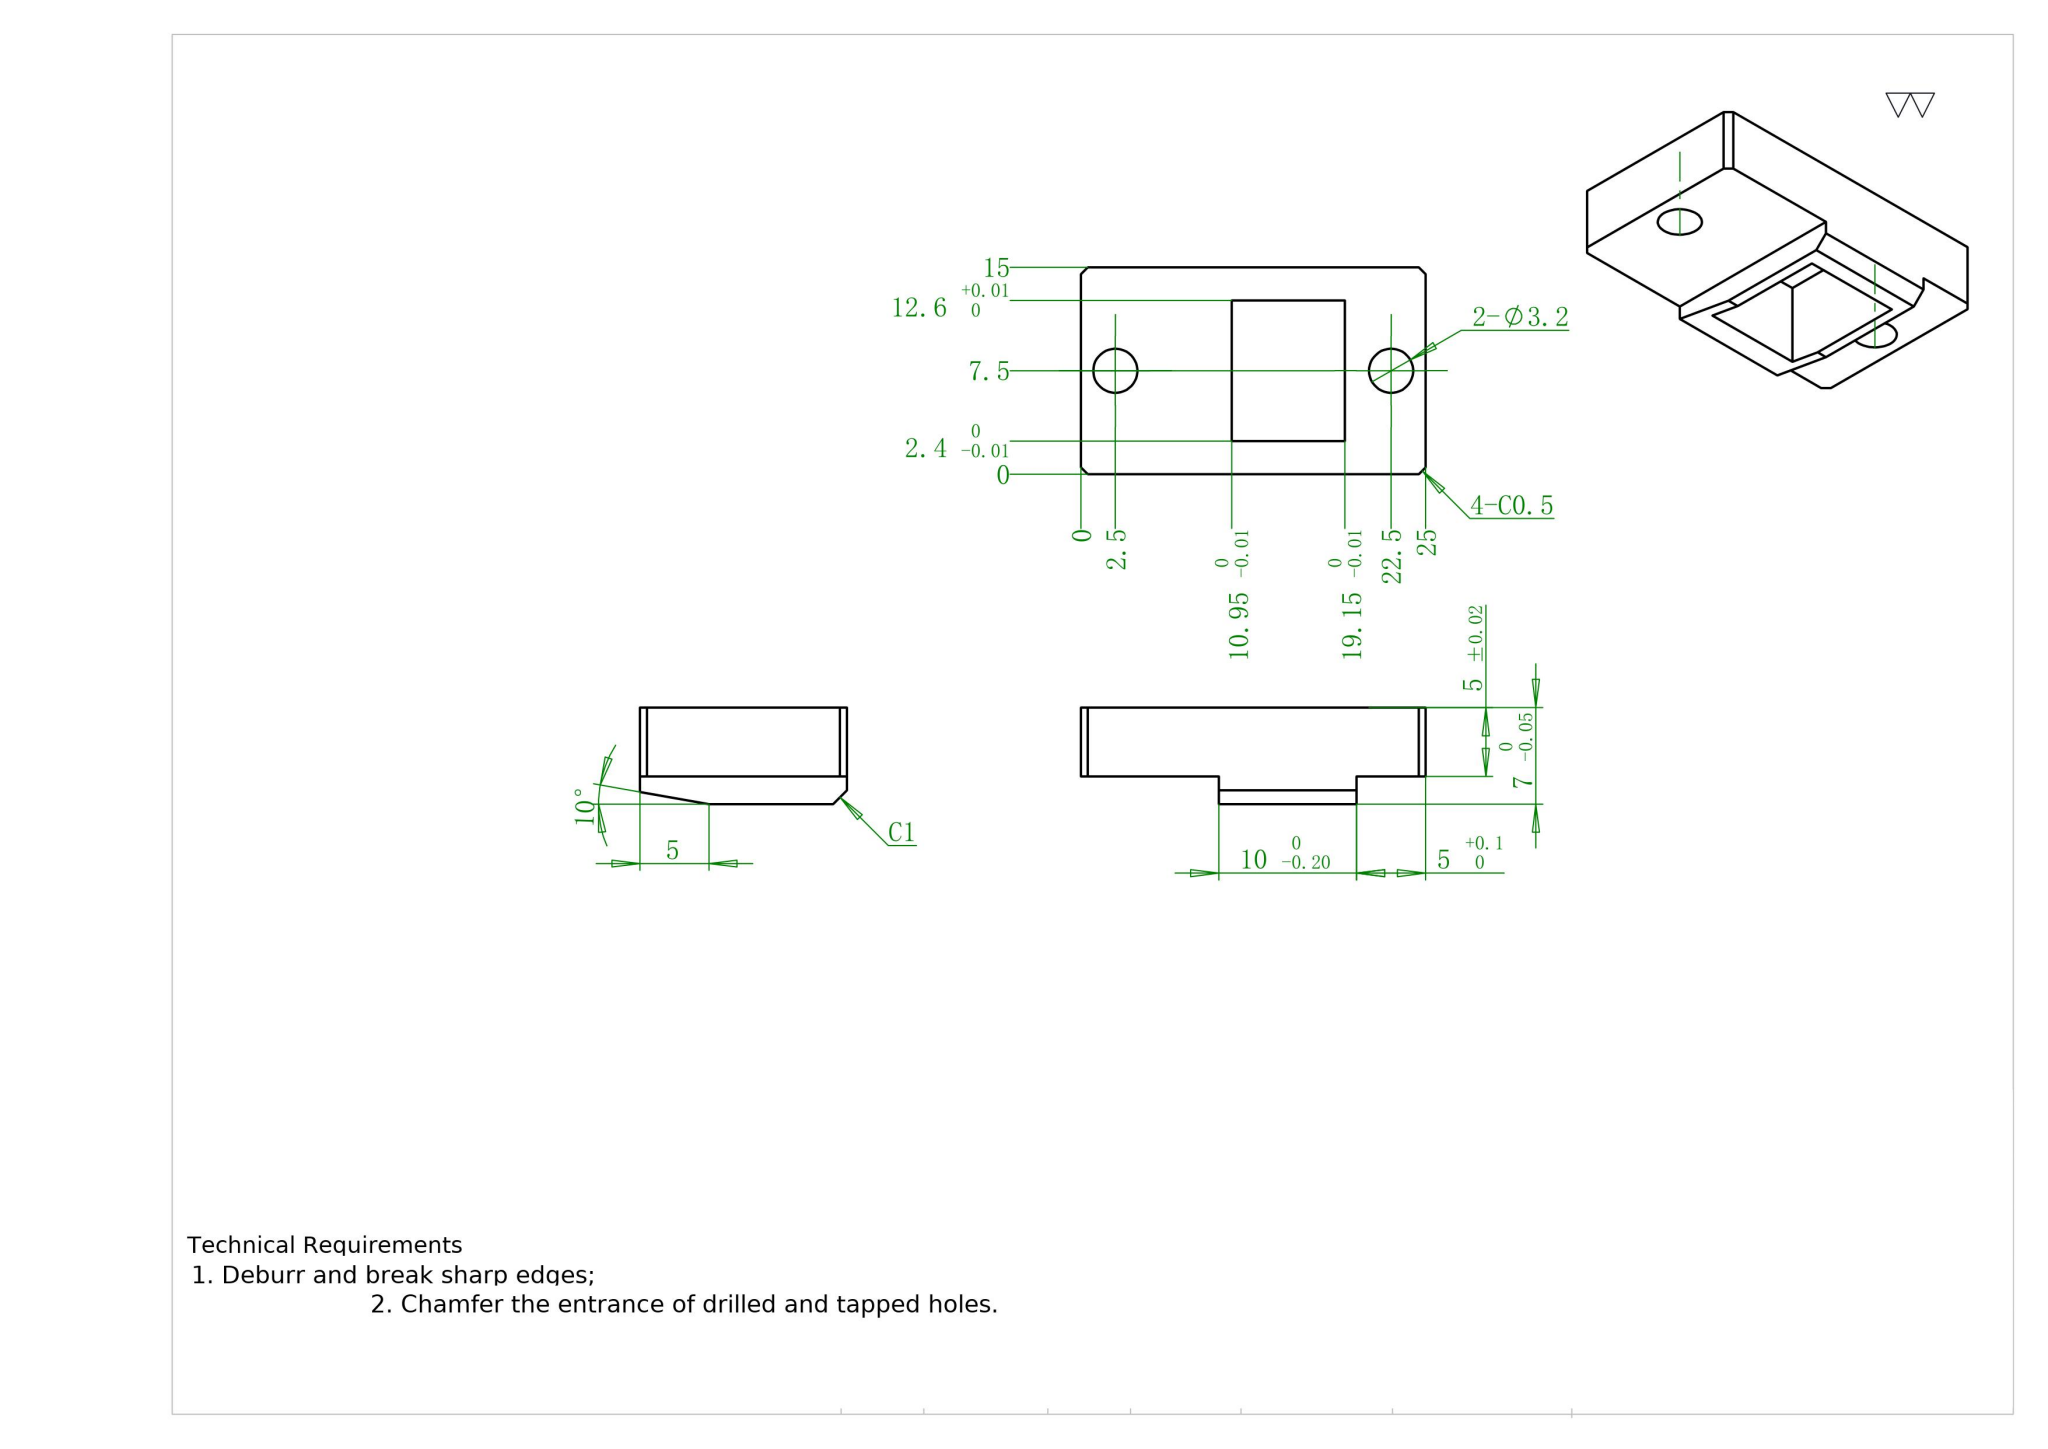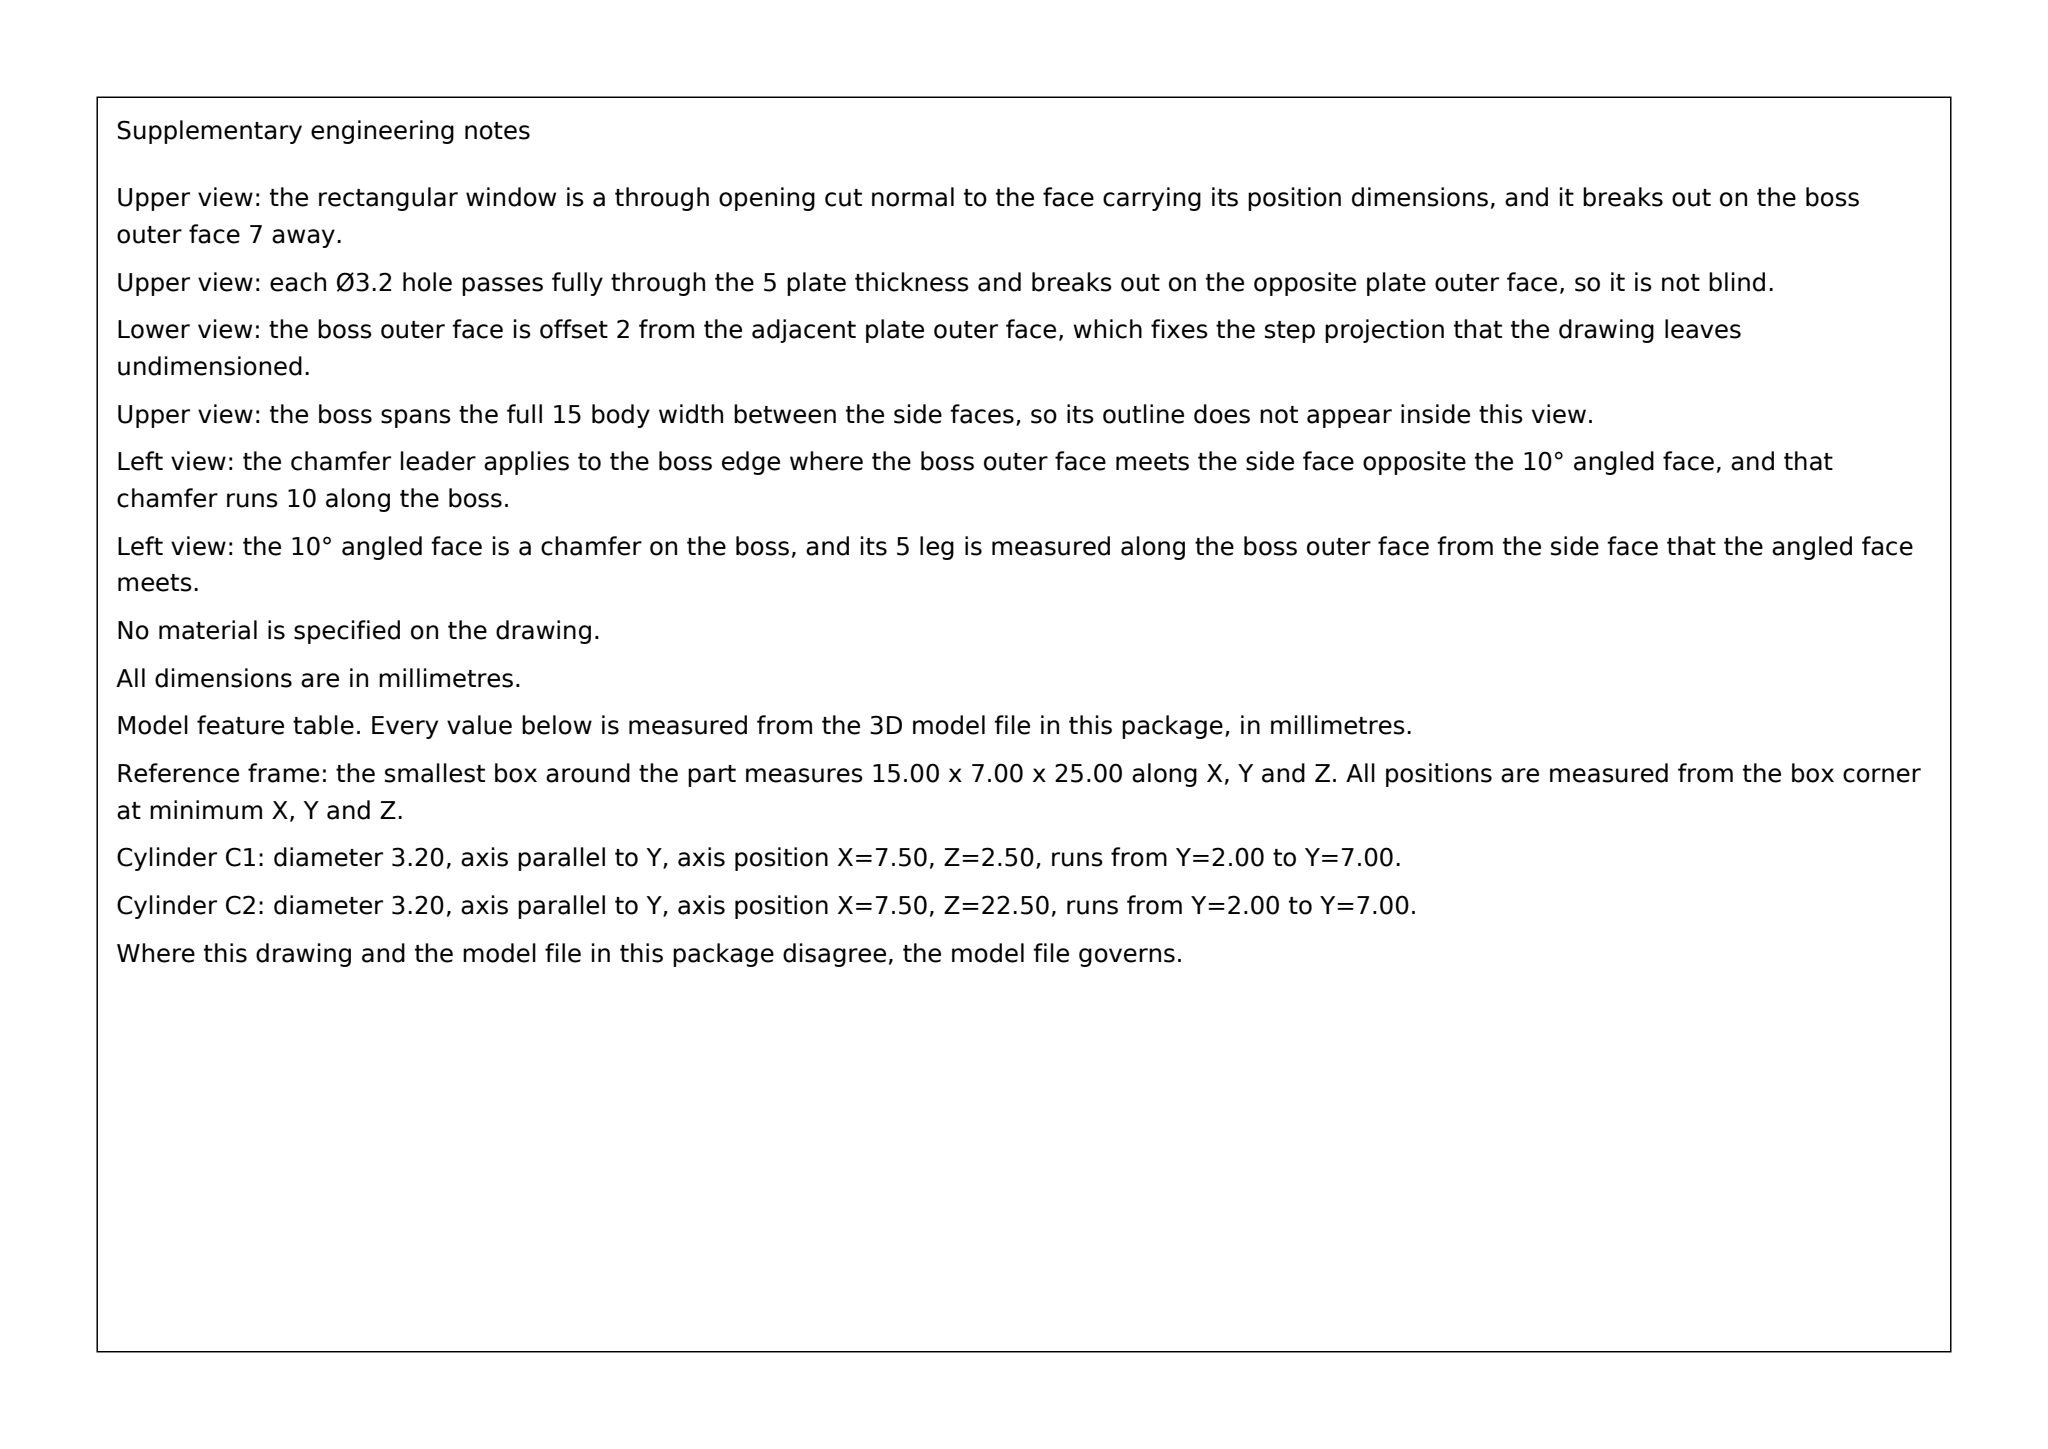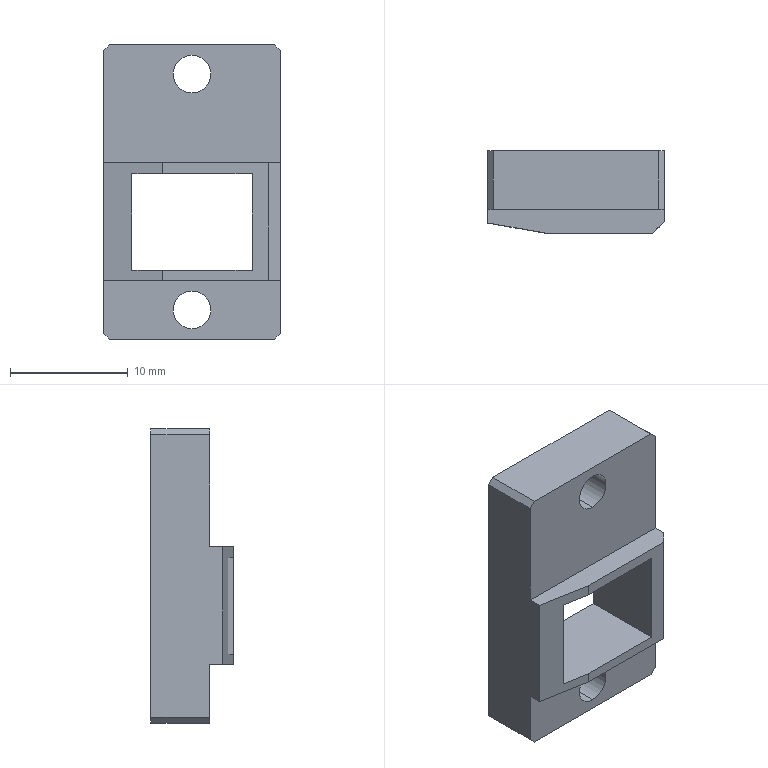Part | SolidWorks | mm | 1 solid | 24 faces | box 15 x 7 x 25 mm | volume 1484 mm3 | plane 20 | cylinder 4 | commonest cylinder face diameters 3.2 x4
Drawing notes:
2-Ø3.2 DP 5 (BLIND, FROM TOP FACE) | from the solid: cylinders dia 3.2, axis y, length 5.0 at z=2.5 and z=22.5, bbox y=7.0 so holes start at top face y=7 and end at y=2.0 (y-plane 2.0 count 2)
STEP:
#1=CARTESIAN_POINT('',(0.,-2.5,0.9));
#2=VERTEX_POINT('',#1);
#3=CARTESIAN_POINT('',(0.,-2.5,4.1));
#4=VERTEX_POINT('',#3);
#5=CARTESIAN_POINT('',(0.,-2.5,2.5));
#6=DIRECTION('',(0.,1.,0.));
#7=DIRECTION('',(0.,0.,1.));
#8=AXIS2_PLACEMENT_3D('',#5,#6,#7);
#9=CIRCLE('',#8,1.6);
#10=EDGE_CURVE('',#2,#4,#9,.T.);
#11=ORIENTED_EDGE('',*,*,#10,.F.);
#12=CARTESIAN_POINT('',(0.,2.5,0.9));
#13=VERTEX_POINT('',#12);
#14=CARTESIAN_POINT('',(0.,2.5,0.9));
#15=DIRECTION('',(0.,1.,0.));
#16=VECTOR('',#15,1000.);
#17=LINE('',#14,#16);
#18=EDGE_CURVE('',#2,#13,#17,.T.);
#19=ORIENTED_EDGE('',*,*,#18,.T.);
#20=CARTESIAN_POINT('',(0.,2.5,4.1));
#21=VERTEX_POINT('',#20);
#22=CARTESIAN_POINT('',(0.,2.5,2.5));
#23=DIRECTION('',(0.,1.,0.));
#24=DIRECTION('',(0.,0.,1.));
#25=AXIS2_PLACEMENT_3D('',#22,#23,#24);
#26=CIRCLE('',#25,1.6);
#27=EDGE_CURVE('',#13,#21,#26,.T.);
#28=ORIENTED_EDGE('',*,*,#27,.T.);
#29=CARTESIAN_POINT('',(0.,2.5,4.1));
#30=DIRECTION('',(0.,1.,0.));
#31=VECTOR('',#30,1000.);
#32=LINE('',#29,#31);
#33=EDGE_CURVE('',#4,#21,#32,.T.);
#34=ORIENTED_EDGE('',*,*,#33,.F.);
#35=EDGE_LOOP('',(#11,#19,#28,#34));
#36=FACE_OUTER_BOUND('',#35,.T.);
#37=CARTESIAN_POINT('',(0.,2.5,2.5));
#38=DIRECTION('',(0.,1.,0.));
#39=DIRECTION('',(0.,0.,1.));
#40=AXIS2_PLACEMENT_3D('',#37,#38,#39);
#41=CYLINDRICAL_SURFACE('',#40,1.6);
#42=ADVANCED_FACE('',(#36),#41,.F.);
#43=CARTESIAN_POINT('',(0.,-2.5,20.9));
#44=VERTEX_POINT('',#43);
#45=CARTESIAN_POINT('',(0.,-2.5,24.1));
#46=VERTEX_POINT('',#45);
#47=CARTESIAN_POINT('',(0.,-2.5,22.5));
#48=DIRECTION('',(0.,1.,0.));
#49=DIRECTION('',(0.,0.,1.));
#50=AXIS2_PLACEMENT_3D('',#47,#48,#49);
#51=CIRCLE('',#50,1.6);
#52=EDGE_CURVE('',#44,#46,#51,.T.);
#53=ORIENTED_EDGE('',*,*,#52,.F.);
#54=CARTESIAN_POINT('',(0.,2.5,20.9));
#55=VERTEX_POINT('',#54);
#56=CARTESIAN_POINT('',(0.,2.5,20.9));
#57=DIRECTION('',(0.,1.,0.));
#58=VECTOR('',#57,1000.);
#59=LINE('',#56,#58);
#60=EDGE_CURVE('',#44,#55,#59,.T.);
#61=ORIENTED_EDGE('',*,*,#60,.T.);
#62=CARTESIAN_POINT('',(0.,2.5,24.1));
#63=VERTEX_POINT('',#62);
#64=CARTESIAN_POINT('',(0.,2.5,22.5));
#65=DIRECTION('',(0.,1.,0.));
#66=DIRECTION('',(0.,0.,1.));
#67=AXIS2_PLACEMENT_3D('',#64,#65,#66);
#68=CIRCLE('',#67,1.6);
#69=EDGE_CURVE('',#55,#63,#68,.T.);
#70=ORIENTED_EDGE('',*,*,#69,.T.);
#71=CARTESIAN_POINT('',(0.,2.5,24.1));
#72=DIRECTION('',(0.,1.,0.));
#73=VECTOR('',#72,1000.);
#74=LINE('',#71,#73);
#75=EDGE_CURVE('',#46,#63,#74,.T.);
#76=ORIENTED_EDGE('',*,*,#75,.F.);
#77=EDGE_LOOP('',(#53,#61,#70,#76));
#78=FACE_OUTER_BOUND('',#77,.T.);
#79=CARTESIAN_POINT('',(0.,2.5,22.5));
#80=DIRECTION('',(0.,1.,0.));
#81=DIRECTION('',(0.,0.,1.));
#82=AXIS2_PLACEMENT_3D('',#79,#80,#81);
#83=CYLINDRICAL_SURFACE('',#82,1.6);
#84=ADVANCED_FACE('',(#78),#83,.F.);
#85=CARTESIAN_POINT('',(0.,-2.5,2.5));
#86=DIRECTION('',(0.,1.,0.));
#87=DIRECTION('',(0.,0.,1.));
#88=AXIS2_PLACEMENT_3D('',#85,#86,#87);
#89=CIRCLE('',#88,1.6);
#90=EDGE_CURVE('',#4,#2,#89,.T.);
#91=ORIENTED_EDGE('',*,*,#90,.T.);
#92=ORIENTED_EDGE('',*,*,#10,.T.);
#93=EDGE_LOOP('',(#91,#92));
#94=FACE_BOUND('',#93,.T.);
#95=CARTESIAN_POINT('',(-7.,-2.5,0.));
#96=VERTEX_POINT('',#95);
#97=CARTESIAN_POINT('',(7.,-2.5,0.));
#98=VERTEX_POINT('',#97);
#99=CARTESIAN_POINT('',(-7.5,-2.5,0.));
#100=DIRECTION('',(1.,0.,0.));
#101=VECTOR('',#100,1000.);
#102=LINE('',#99,#101);
#103=EDGE_CURVE('',#96,#98,#102,.T.);
#104=ORIENTED_EDGE('',*,*,#103,.T.);
#105=CARTESIAN_POINT('',(7.5,-2.5,0.5));
#106=VERTEX_POINT('',#105);
#107=CARTESIAN_POINT('',(7.5,-2.5,0.5));
#108=DIRECTION('',(0.7071,0.,0.7071));
#109=VECTOR('',#108,1000.);
#110=LINE('',#107,#109);
#111=EDGE_CURVE('',#98,#106,#110,.T.);
#112=ORIENTED_EDGE('',*,*,#111,.T.);
#113=CARTESIAN_POINT('',(7.5,-2.5,5.));
#114=VERTEX_POINT('',#113);
#115=CARTESIAN_POINT('',(7.5,-2.5,25.));
#116=DIRECTION('',(0.,0.,-1.));
#117=VECTOR('',#116,1000.);
#118=LINE('',#115,#117);
#119=EDGE_CURVE('',#114,#106,#118,.T.);
#120=ORIENTED_EDGE('',*,*,#119,.F.);
#121=CARTESIAN_POINT('',(-7.5,-2.5,5.));
#122=VERTEX_POINT('',#121);
#123=CARTESIAN_POINT('',(7.5,-2.5,5.));
#124=DIRECTION('',(1.,0.,0.));
#125=VECTOR('',#124,1000.);
#126=LINE('',#123,#125);
#127=EDGE_CURVE('',#122,#114,#126,.T.);
#128=ORIENTED_EDGE('',*,*,#127,.F.);
#129=CARTESIAN_POINT('',(-7.5,-2.5,0.5));
#130=VERTEX_POINT('',#129);
#131=CARTESIAN_POINT('',(-7.5,-2.5,25.));
#132=DIRECTION('',(0.,0.,-1.));
#133=VECTOR('',#132,1000.);
#134=LINE('',#131,#133);
#135=EDGE_CURVE('',#122,#130,#134,.T.);
#136=ORIENTED_EDGE('',*,*,#135,.T.);
#137=CARTESIAN_POINT('',(-7.5,-2.5,0.5));
#138=DIRECTION('',(0.7071,0.,-0.7071));
#139=VECTOR('',#138,1000.);
#140=LINE('',#137,#139);
#141=EDGE_CURVE('',#130,#96,#140,.T.);
#142=ORIENTED_EDGE('',*,*,#141,.T.);
#143=EDGE_LOOP('',(#104,#112,#120,#128,#136,#142));
#144=FACE_OUTER_BOUND('',#143,.T.);
#145=CARTESIAN_POINT('',(-7.5,-2.5,25.));
#146=DIRECTION('',(0.,1.,0.));
#147=DIRECTION('',(0.,0.,1.));
#148=AXIS2_PLACEMENT_3D('',#145,#146,#147);
#149=PLANE('',#148);
#150=ADVANCED_FACE('',(#94,#144),#149,.F.);
#151=CARTESIAN_POINT('',(0.,-2.5,22.5));
#152=DIRECTION('',(0.,1.,0.));
#153=DIRECTION('',(0.,0.,1.));
#154=AXIS2_PLACEMENT_3D('',#151,#152,#153);
#155=CIRCLE('',#154,1.6);
#156=EDGE_CURVE('',#46,#44,#155,.T.);
#157=ORIENTED_EDGE('',*,*,#156,.T.);
#158=ORIENTED_EDGE('',*,*,#52,.T.);
#159=EDGE_LOOP('',(#157,#158));
#160=FACE_BOUND('',#159,.T.);
#161=CARTESIAN_POINT('',(-7.,-2.5,25.));
#162=VERTEX_POINT('',#161);
#163=CARTESIAN_POINT('',(7.,-2.5,25.));
#164=VERTEX_POINT('',#163);
#165=CARTESIAN_POINT('',(-7.5,-2.5,25.));
#166=DIRECTION('',(1.,0.,0.));
#167=VECTOR('',#166,1000.);
#168=LINE('',#165,#167);
#169=EDGE_CURVE('',#162,#164,#168,.T.);
#170=ORIENTED_EDGE('',*,*,#169,.F.);
#171=CARTESIAN_POINT('',(-7.5,-2.5,24.5));
#172=VERTEX_POINT('',#171);
#173=CARTESIAN_POINT('',(-7.,-2.5,25.));
#174=DIRECTION('',(-0.7071,0.,-0.7071));
#175=VECTOR('',#174,1000.);
#176=LINE('',#173,#175);
#177=EDGE_CURVE('',#162,#172,#176,.T.);
#178=ORIENTED_EDGE('',*,*,#177,.T.);
#179=CARTESIAN_POINT('',(-7.5,-2.5,15.));
#180=VERTEX_POINT('',#179);
#181=CARTESIAN_POINT('',(-7.5,-2.5,25.));
#182=DIRECTION('',(0.,0.,-1.));
#183=VECTOR('',#182,1000.);
#184=LINE('',#181,#183);
#185=EDGE_CURVE('',#172,#180,#184,.T.);
#186=ORIENTED_EDGE('',*,*,#185,.T.);
#187=CARTESIAN_POINT('',(7.5,-2.5,15.));
#188=VERTEX_POINT('',#187);
#189=CARTESIAN_POINT('',(7.5,-2.5,15.));
#190=DIRECTION('',(-1.,0.,-0.));
#191=VECTOR('',#190,1000.);
#192=LINE('',#189,#191);
#193=EDGE_CURVE('',#188,#180,#192,.T.);
#194=ORIENTED_EDGE('',*,*,#193,.F.);
#195=CARTESIAN_POINT('',(7.5,-2.5,24.5));
#196=VERTEX_POINT('',#195);
#197=CARTESIAN_POINT('',(7.5,-2.5,25.));
#198=DIRECTION('',(0.,0.,-1.));
#199=VECTOR('',#198,1000.);
#200=LINE('',#197,#199);
#201=EDGE_CURVE('',#196,#188,#200,.T.);
#202=ORIENTED_EDGE('',*,*,#201,.F.);
#203=CARTESIAN_POINT('',(7.,-2.5,25.));
#204=DIRECTION('',(-0.7071,0.,0.7071));
#205=VECTOR('',#204,1000.);
#206=LINE('',#203,#205);
#207=EDGE_CURVE('',#196,#164,#206,.T.);
#208=ORIENTED_EDGE('',*,*,#207,.T.);
#209=EDGE_LOOP('',(#170,#178,#186,#194,#202,#208));
#210=FACE_OUTER_BOUND('',#209,.T.);
#211=CARTESIAN_POINT('',(-7.5,-2.5,25.));
#212=DIRECTION('',(0.,1.,0.));
#213=DIRECTION('',(0.,0.,1.));
#214=AXIS2_PLACEMENT_3D('',#211,#212,#213);
#215=PLANE('',#214);
#216=ADVANCED_FACE('',(#160,#210),#215,.F.);
#217=CARTESIAN_POINT('',(7.5,-3.5,15.));
#218=VERTEX_POINT('',#217);
#219=CARTESIAN_POINT('',(7.5,-4.5,15.));
#220=DIRECTION('',(0.,1.,0.));
#221=VECTOR('',#220,1000.);
#222=LINE('',#219,#221);
#223=EDGE_CURVE('',#218,#188,#222,.T.);
#224=ORIENTED_EDGE('',*,*,#223,.F.);
#225=CARTESIAN_POINT('',(7.5,-3.5,5.));
#226=VERTEX_POINT('',#225);
#227=CARTESIAN_POINT('',(7.5,-3.5,5.));
#228=DIRECTION('',(0.,0.,-1.));
#229=VECTOR('',#228,1000.);
#230=LINE('',#227,#229);
#231=EDGE_CURVE('',#218,#226,#230,.T.);
#232=ORIENTED_EDGE('',*,*,#231,.T.);
#233=CARTESIAN_POINT('',(7.5,-4.5,5.));
#234=DIRECTION('',(0.,1.,0.));
#235=VECTOR('',#234,1000.);
#236=LINE('',#233,#235);
#237=EDGE_CURVE('',#226,#114,#236,.T.);
#238=ORIENTED_EDGE('',*,*,#237,.T.);
#239=ORIENTED_EDGE('',*,*,#119,.T.);
#240=CARTESIAN_POINT('',(7.5,2.5,0.5));
#241=VERTEX_POINT('',#240);
#242=CARTESIAN_POINT('',(7.5,2.5,0.5));
#243=DIRECTION('',(-0.,1.,0.));
#244=VECTOR('',#243,1000.);
#245=LINE('',#242,#244);
#246=EDGE_CURVE('',#106,#241,#245,.T.);
#247=ORIENTED_EDGE('',*,*,#246,.T.);
#248=CARTESIAN_POINT('',(7.5,2.5,24.5));
#249=VERTEX_POINT('',#248);
#250=CARTESIAN_POINT('',(7.5,2.5,25.));
#251=DIRECTION('',(0.,0.,-1.));
#252=VECTOR('',#251,1000.);
#253=LINE('',#250,#252);
#254=EDGE_CURVE('',#249,#241,#253,.T.);
#255=ORIENTED_EDGE('',*,*,#254,.F.);
#256=CARTESIAN_POINT('',(7.5,-2.5,24.5));
#257=DIRECTION('',(0.,-1.,0.));
#258=VECTOR('',#257,1000.);
#259=LINE('',#256,#258);
#260=EDGE_CURVE('',#249,#196,#259,.T.);
#261=ORIENTED_EDGE('',*,*,#260,.T.);
#262=ORIENTED_EDGE('',*,*,#201,.T.);
#263=EDGE_LOOP('',(#224,#232,#238,#239,#247,#255,#261,#262));
#264=FACE_OUTER_BOUND('',#263,.T.);
#265=CARTESIAN_POINT('',(7.5,2.5,25.));
#266=DIRECTION('',(-1.,-0.,0.));
#267=DIRECTION('',(0.,-1.,0.));
#268=AXIS2_PLACEMENT_3D('',#265,#266,#267);
#269=PLANE('',#268);
#270=ADVANCED_FACE('',(#264),#269,.F.);
#271=CARTESIAN_POINT('',(0.,2.5,2.5));
#272=DIRECTION('',(0.,1.,0.));
#273=DIRECTION('',(0.,0.,1.));
#274=AXIS2_PLACEMENT_3D('',#271,#272,#273);
#275=CIRCLE('',#274,1.6);
#276=EDGE_CURVE('',#21,#13,#275,.T.);
#277=ORIENTED_EDGE('',*,*,#276,.F.);
#278=ORIENTED_EDGE('',*,*,#27,.F.);
#279=EDGE_LOOP('',(#277,#278));
#280=FACE_BOUND('',#279,.T.);
#281=CARTESIAN_POINT('',(0.,2.5,22.5));
#282=DIRECTION('',(0.,1.,0.));
#283=DIRECTION('',(0.,0.,1.));
#284=AXIS2_PLACEMENT_3D('',#281,#282,#283);
#285=CIRCLE('',#284,1.6);
#286=EDGE_CURVE('',#63,#55,#285,.T.);
#287=ORIENTED_EDGE('',*,*,#286,.F.);
#288=ORIENTED_EDGE('',*,*,#69,.F.);
#289=EDGE_LOOP('',(#287,#288));
#290=FACE_BOUND('',#289,.T.);
#291=CARTESIAN_POINT('',(-5.1,2.5,14.05));
#292=VERTEX_POINT('',#291);
#293=CARTESIAN_POINT('',(5.1,2.5,14.05));
#294=VERTEX_POINT('',#293);
#295=CARTESIAN_POINT('',(5.1,2.5,14.05));
#296=DIRECTION('',(1.,0.,-0.));
#297=VECTOR('',#296,1000.);
#298=LINE('',#295,#297);
#299=EDGE_CURVE('',#292,#294,#298,.T.);
#300=ORIENTED_EDGE('',*,*,#299,.F.);
#301=CARTESIAN_POINT('',(-5.1,2.5,5.85));
#302=VERTEX_POINT('',#301);
#303=CARTESIAN_POINT('',(-5.1,2.5,5.85));
#304=DIRECTION('',(0.,0.,1.));
#305=VECTOR('',#304,1000.);
#306=LINE('',#303,#305);
#307=EDGE_CURVE('',#302,#292,#306,.T.);
#308=ORIENTED_EDGE('',*,*,#307,.F.);
#309=CARTESIAN_POINT('',(5.1,2.5,5.85));
#310=VERTEX_POINT('',#309);
#311=CARTESIAN_POINT('',(5.1,2.5,5.85));
#312=DIRECTION('',(-1.,0.,0.));
#313=VECTOR('',#312,1000.);
#314=LINE('',#311,#313);
#315=EDGE_CURVE('',#310,#302,#314,.T.);
#316=ORIENTED_EDGE('',*,*,#315,.F.);
#317=CARTESIAN_POINT('',(5.1,2.5,5.85));
#318=DIRECTION('',(-0.,0.,-1.));
#319=VECTOR('',#318,1000.);
#320=LINE('',#317,#319);
#321=EDGE_CURVE('',#294,#310,#320,.T.);
#322=ORIENTED_EDGE('',*,*,#321,.F.);
#323=EDGE_LOOP('',(#300,#308,#316,#322));
#324=FACE_BOUND('',#323,.T.);
#325=ORIENTED_EDGE('',*,*,#254,.T.);
#326=CARTESIAN_POINT('',(7.,2.5,0.));
#327=VERTEX_POINT('',#326);
#328=CARTESIAN_POINT('',(7.5,2.5,0.5));
#329=DIRECTION('',(-0.7071,0.,-0.7071));
#330=VECTOR('',#329,1000.);
#331=LINE('',#328,#330);
#332=EDGE_CURVE('',#241,#327,#331,.T.);
#333=ORIENTED_EDGE('',*,*,#332,.T.);
#334=CARTESIAN_POINT('',(-7.,2.5,-0.));
#335=VERTEX_POINT('',#334);
#336=CARTESIAN_POINT('',(-7.5,2.5,0.));
#337=DIRECTION('',(-1.,0.,0.));
#338=VECTOR('',#337,1000.);
#339=LINE('',#336,#338);
#340=EDGE_CURVE('',#327,#335,#339,.T.);
#341=ORIENTED_EDGE('',*,*,#340,.T.);
#342=CARTESIAN_POINT('',(-7.5,2.5,0.5));
#343=VERTEX_POINT('',#342);
#344=CARTESIAN_POINT('',(-7.5,2.5,0.5));
#345=DIRECTION('',(-0.7071,0.,0.7071));
#346=VECTOR('',#345,1000.);
#347=LINE('',#344,#346);
#348=EDGE_CURVE('',#335,#343,#347,.T.);
#349=ORIENTED_EDGE('',*,*,#348,.T.);
#350=CARTESIAN_POINT('',(-7.5,2.5,24.5));
#351=VERTEX_POINT('',#350);
#352=CARTESIAN_POINT('',(-7.5,2.5,25.));
#353=DIRECTION('',(0.,0.,-1.));
#354=VECTOR('',#353,1000.);
#355=LINE('',#352,#354);
#356=EDGE_CURVE('',#351,#343,#355,.T.);
#357=ORIENTED_EDGE('',*,*,#356,.F.);
#358=CARTESIAN_POINT('',(-7.,2.5,25.));
#359=VERTEX_POINT('',#358);
#360=CARTESIAN_POINT('',(-7.,2.5,25.));
#361=DIRECTION('',(0.7071,0.,0.7071));
#362=VECTOR('',#361,1000.);
#363=LINE('',#360,#362);
#364=EDGE_CURVE('',#351,#359,#363,.T.);
#365=ORIENTED_EDGE('',*,*,#364,.T.);
#366=CARTESIAN_POINT('',(7.,2.5,25.));
#367=VERTEX_POINT('',#366);
#368=CARTESIAN_POINT('',(-7.5,2.5,25.));
#369=DIRECTION('',(-1.,0.,0.));
#370=VECTOR('',#369,1000.);
#371=LINE('',#368,#370);
#372=EDGE_CURVE('',#367,#359,#371,.T.);
#373=ORIENTED_EDGE('',*,*,#372,.F.);
#374=CARTESIAN_POINT('',(7.,2.5,25.));
#375=DIRECTION('',(0.7071,0.,-0.7071));
#376=VECTOR('',#375,1000.);
#377=LINE('',#374,#376);
#378=EDGE_CURVE('',#367,#249,#377,.T.);
#379=ORIENTED_EDGE('',*,*,#378,.T.);
#380=EDGE_LOOP('',(#325,#333,#341,#349,#357,#365,#373,#379));
#381=FACE_OUTER_BOUND('',#380,.T.);
#382=CARTESIAN_POINT('',(-7.5,2.5,25.));
#383=DIRECTION('',(0.,-1.,0.));
#384=DIRECTION('',(0.,0.,-1.));
#385=AXIS2_PLACEMENT_3D('',#382,#383,#384);
#386=PLANE('',#385);
#387=ADVANCED_FACE('',(#280,#290,#324,#381),#386,.F.);
#388=ORIENTED_EDGE('',*,*,#356,.T.);
#389=CARTESIAN_POINT('',(-7.5,2.5,0.5));
#390=DIRECTION('',(0.,-1.,0.));
#391=VECTOR('',#390,1000.);
#392=LINE('',#389,#391);
#393=EDGE_CURVE('',#343,#130,#392,.T.);
#394=ORIENTED_EDGE('',*,*,#393,.T.);
#395=ORIENTED_EDGE('',*,*,#135,.F.);
#396=CARTESIAN_POINT('',(-7.5,-3.618,5.));
#397=VERTEX_POINT('',#396);
#398=CARTESIAN_POINT('',(-7.5,-4.5,5.));
#399=DIRECTION('',(0.,1.,0.));
#400=VECTOR('',#399,1000.);
#401=LINE('',#398,#400);
#402=EDGE_CURVE('',#397,#122,#401,.T.);
#403=ORIENTED_EDGE('',*,*,#402,.F.);
#404=CARTESIAN_POINT('',(-7.5,-3.618,15.));
#405=VERTEX_POINT('',#404);
#406=CARTESIAN_POINT('',(-7.5,-3.618,15.));
#407=DIRECTION('',(0.,0.,1.));
#408=VECTOR('',#407,1000.);
#409=LINE('',#406,#408);
#410=EDGE_CURVE('',#397,#405,#409,.T.);
#411=ORIENTED_EDGE('',*,*,#410,.T.);
#412=CARTESIAN_POINT('',(-7.5,-4.5,15.));
#413=DIRECTION('',(0.,1.,0.));
#414=VECTOR('',#413,1000.);
#415=LINE('',#412,#414);
#416=EDGE_CURVE('',#405,#180,#415,.T.);
#417=ORIENTED_EDGE('',*,*,#416,.T.);
#418=ORIENTED_EDGE('',*,*,#185,.F.);
#419=CARTESIAN_POINT('',(-7.5,2.5,24.5));
#420=DIRECTION('',(-0.,1.,0.));
#421=VECTOR('',#420,1000.);
#422=LINE('',#419,#421);
#423=EDGE_CURVE('',#172,#351,#422,.T.);
#424=ORIENTED_EDGE('',*,*,#423,.T.);
#425=EDGE_LOOP('',(#388,#394,#395,#403,#411,#417,#418,#424));
#426=FACE_OUTER_BOUND('',#425,.T.);
#427=CARTESIAN_POINT('',(-7.5,2.5,25.));
#428=DIRECTION('',(1.,0.,0.));
#429=DIRECTION('',(-0.,1.,0.));
#430=AXIS2_PLACEMENT_3D('',#427,#428,#429);
#431=PLANE('',#430);
#432=ADVANCED_FACE('',(#426),#431,.F.);
#433=ORIENTED_EDGE('',*,*,#372,.T.);
#434=CARTESIAN_POINT('',(-7.,-2.5,25.));
#435=DIRECTION('',(0.,-1.,0.));
#436=VECTOR('',#435,1000.);
#437=LINE('',#434,#436);
#438=EDGE_CURVE('',#359,#162,#437,.T.);
#439=ORIENTED_EDGE('',*,*,#438,.T.);
#440=ORIENTED_EDGE('',*,*,#169,.T.);
#441=CARTESIAN_POINT('',(7.,2.5,25.));
#442=DIRECTION('',(-0.,1.,0.));
#443=VECTOR('',#442,1000.);
#444=LINE('',#441,#443);
#445=EDGE_CURVE('',#164,#367,#444,.T.);
#446=ORIENTED_EDGE('',*,*,#445,.T.);
#447=EDGE_LOOP('',(#433,#439,#440,#446));
#448=FACE_OUTER_BOUND('',#447,.T.);
#449=CARTESIAN_POINT('',(0.,0.,25.));
#450=DIRECTION('',(0.,0.,1.));
#451=DIRECTION('',(1.,0.,0.));
#452=AXIS2_PLACEMENT_3D('',#449,#450,#451);
#453=PLANE('',#452);
#454=ADVANCED_FACE('',(#448),#453,.T.);
#455=ORIENTED_EDGE('',*,*,#340,.F.);
#456=CARTESIAN_POINT('',(7.,0.,0.));
#457=DIRECTION('',(0.,-1.,0.));
#458=VECTOR('',#457,1000.);
#459=LINE('',#456,#458);
#460=EDGE_CURVE('',#327,#98,#459,.T.);
#461=ORIENTED_EDGE('',*,*,#460,.T.);
#462=ORIENTED_EDGE('',*,*,#103,.F.);
#463=CARTESIAN_POINT('',(-7.,-0.,0.));
#464=DIRECTION('',(-0.,1.,0.));
#465=VECTOR('',#464,1000.);
#466=LINE('',#463,#465);
#467=EDGE_CURVE('',#96,#335,#466,.T.);
#468=ORIENTED_EDGE('',*,*,#467,.T.);
#469=EDGE_LOOP('',(#455,#461,#462,#468));
#470=FACE_OUTER_BOUND('',#469,.T.);
#471=CARTESIAN_POINT('',(0.,0.,0.));
#472=DIRECTION('',(0.,0.,1.));
#473=DIRECTION('',(1.,0.,0.));
#474=AXIS2_PLACEMENT_3D('',#471,#472,#473);
#475=PLANE('',#474);
#476=ADVANCED_FACE('',(#470),#475,.F.);
#477=CARTESIAN_POINT('',(6.5,-4.5,15.));
#478=VERTEX_POINT('',#477);
#479=CARTESIAN_POINT('',(-2.5,-4.5,15.));
#480=VERTEX_POINT('',#479);
#481=CARTESIAN_POINT('',(7.5,-4.5,15.));
#482=DIRECTION('',(-1.,0.,-0.));
#483=VECTOR('',#482,1000.);
#484=LINE('',#481,#483);
#485=EDGE_CURVE('',#478,#480,#484,.T.);
#486=ORIENTED_EDGE('',*,*,#485,.F.);
#487=CARTESIAN_POINT('',(6.5,-4.5,15.));
#488=DIRECTION('',(0.7071,0.7071,0.));
#489=VECTOR('',#488,1000.);
#490=LINE('',#487,#489);
#491=EDGE_CURVE('',#478,#218,#490,.T.);
#492=ORIENTED_EDGE('',*,*,#491,.T.);
#493=ORIENTED_EDGE('',*,*,#223,.T.);
#494=ORIENTED_EDGE('',*,*,#193,.T.);
#495=ORIENTED_EDGE('',*,*,#416,.F.);
#496=CARTESIAN_POINT('',(-2.5,-4.5,15.));
#497=DIRECTION('',(0.9848,-0.1736,0.));
#498=VECTOR('',#497,1000.);
#499=LINE('',#496,#498);
#500=EDGE_CURVE('',#405,#480,#499,.T.);
#501=ORIENTED_EDGE('',*,*,#500,.T.);
#502=EDGE_LOOP('',(#486,#492,#493,#494,#495,#501));
#503=FACE_OUTER_BOUND('',#502,.T.);
#504=CARTESIAN_POINT('',(7.5,-4.5,15.));
#505=DIRECTION('',(0.,0.,-1.));
#506=DIRECTION('',(-1.,0.,-0.));
#507=AXIS2_PLACEMENT_3D('',#504,#505,#506);
#508=PLANE('',#507);
#509=ADVANCED_FACE('',(#503),#508,.F.);
#510=ORIENTED_EDGE('',*,*,#237,.F.);
#511=CARTESIAN_POINT('',(6.5,-4.5,5.));
#512=VERTEX_POINT('',#511);
#513=CARTESIAN_POINT('',(6.5,-4.5,5.));
#514=DIRECTION('',(-0.7071,-0.7071,-0.));
#515=VECTOR('',#514,1000.);
#516=LINE('',#513,#515);
#517=EDGE_CURVE('',#226,#512,#516,.T.);
#518=ORIENTED_EDGE('',*,*,#517,.T.);
#519=CARTESIAN_POINT('',(-2.5,-4.5,5.));
#520=VERTEX_POINT('',#519);
#521=CARTESIAN_POINT('',(7.5,-4.5,5.));
#522=DIRECTION('',(1.,0.,0.));
#523=VECTOR('',#522,1000.);
#524=LINE('',#521,#523);
#525=EDGE_CURVE('',#520,#512,#524,.T.);
#526=ORIENTED_EDGE('',*,*,#525,.F.);
#527=CARTESIAN_POINT('',(-2.5,-4.5,5.));
#528=DIRECTION('',(-0.9848,0.1736,-0.));
#529=VECTOR('',#528,1000.);
#530=LINE('',#527,#529);
#531=EDGE_CURVE('',#520,#397,#530,.T.);
#532=ORIENTED_EDGE('',*,*,#531,.T.);
#533=ORIENTED_EDGE('',*,*,#402,.T.);
#534=ORIENTED_EDGE('',*,*,#127,.T.);
#535=EDGE_LOOP('',(#510,#518,#526,#532,#533,#534));
#536=FACE_OUTER_BOUND('',#535,.T.);
#537=CARTESIAN_POINT('',(7.5,-4.5,5.));
#538=DIRECTION('',(-0.,0.,1.));
#539=DIRECTION('',(1.,0.,0.));
#540=AXIS2_PLACEMENT_3D('',#537,#538,#539);
#541=PLANE('',#540);
#542=ADVANCED_FACE('',(#536),#541,.F.);
#543=ORIENTED_EDGE('',*,*,#525,.T.);
#544=CARTESIAN_POINT('',(6.5,-4.5,15.));
#545=DIRECTION('',(0.,0.,1.));
#546=VECTOR('',#545,1000.);
#547=LINE('',#544,#546);
#548=EDGE_CURVE('',#512,#478,#547,.T.);
#549=ORIENTED_EDGE('',*,*,#548,.T.);
#550=ORIENTED_EDGE('',*,*,#485,.T.);
#551=CARTESIAN_POINT('',(-2.5,-4.5,14.05));
#552=VERTEX_POINT('',#551);
#553=CARTESIAN_POINT('',(-2.5,-4.5,5.));
#554=DIRECTION('',(0.,0.,-1.));
#555=VECTOR('',#554,1000.);
#556=LINE('',#553,#555);
#557=EDGE_CURVE('',#480,#552,#556,.T.);
#558=ORIENTED_EDGE('',*,*,#557,.T.);
#559=CARTESIAN_POINT('',(5.1,-4.5,14.05));
#560=VERTEX_POINT('',#559);
#561=CARTESIAN_POINT('',(0.,-4.5,14.05));
#562=DIRECTION('',(-1.,0.,0.));
#563=VECTOR('',#562,1000.);
#564=LINE('',#561,#563);
#565=EDGE_CURVE('',#560,#552,#564,.T.);
#566=ORIENTED_EDGE('',*,*,#565,.F.);
#567=CARTESIAN_POINT('',(5.1,-4.5,5.85));
#568=VERTEX_POINT('',#567);
#569=CARTESIAN_POINT('',(5.1,-4.5,-0.));
#570=DIRECTION('',(0.,0.,1.));
#571=VECTOR('',#570,1000.);
#572=LINE('',#569,#571);
#573=EDGE_CURVE('',#568,#560,#572,.T.);
#574=ORIENTED_EDGE('',*,*,#573,.F.);
#575=CARTESIAN_POINT('',(-2.5,-4.5,5.85));
#576=VERTEX_POINT('',#575);
#577=CARTESIAN_POINT('',(0.,-4.5,5.85));
#578=DIRECTION('',(1.,0.,-0.));
#579=VECTOR('',#578,1000.);
#580=LINE('',#577,#579);
#581=EDGE_CURVE('',#576,#568,#580,.T.);
#582=ORIENTED_EDGE('',*,*,#581,.F.);
#583=CARTESIAN_POINT('',(-2.5,-4.5,5.));
#584=DIRECTION('',(0.,0.,-1.));
#585=VECTOR('',#584,1000.);
#586=LINE('',#583,#585);
#587=EDGE_CURVE('',#576,#520,#586,.T.);
#588=ORIENTED_EDGE('',*,*,#587,.T.);
#589=EDGE_LOOP('',(#543,#549,#550,#558,#566,#574,#582,#588));
#590=FACE_OUTER_BOUND('',#589,.T.);
#591=CARTESIAN_POINT('',(0.,-4.5,0.));
#592=DIRECTION('',(0.,-1.,0.));
#593=DIRECTION('',(0.,0.,-1.));
#594=AXIS2_PLACEMENT_3D('',#591,#592,#593);
#595=PLANE('',#594);
#596=ADVANCED_FACE('',(#590),#595,.T.);
#597=CARTESIAN_POINT('',(-5.1,-4.042,14.05));
#598=VERTEX_POINT('',#597);
#599=CARTESIAN_POINT('',(-5.1,-4.5,14.05));
#600=DIRECTION('',(0.,1.,0.));
#601=VECTOR('',#600,1000.);
#602=LINE('',#599,#601);
#603=EDGE_CURVE('',#598,#292,#602,.T.);
#604=ORIENTED_EDGE('',*,*,#603,.F.);
#605=CARTESIAN_POINT('',(-5.1,-4.042,5.85));
#606=VERTEX_POINT('',#605);
#607=CARTESIAN_POINT('',(-5.1,-4.042,0.));
#608=DIRECTION('',(-0.,0.,-1.));
#609=VECTOR('',#608,1000.);
#610=LINE('',#607,#609);
#611=EDGE_CURVE('',#598,#606,#610,.T.);
#612=ORIENTED_EDGE('',*,*,#611,.T.);
#613=CARTESIAN_POINT('',(-5.1,-4.5,5.85));
#614=DIRECTION('',(0.,1.,0.));
#615=VECTOR('',#614,1000.);
#616=LINE('',#613,#615);
#617=EDGE_CURVE('',#606,#302,#616,.T.);
#618=ORIENTED_EDGE('',*,*,#617,.T.);
#619=ORIENTED_EDGE('',*,*,#307,.T.);
#620=EDGE_LOOP('',(#604,#612,#618,#619));
#621=FACE_OUTER_BOUND('',#620,.T.);
#622=CARTESIAN_POINT('',(-5.1,-4.5,5.85));
#623=DIRECTION('',(-1.,0.,0.));
#624=DIRECTION('',(0.,0.,1.));
#625=AXIS2_PLACEMENT_3D('',#622,#623,#624);
#626=PLANE('',#625);
#627=ADVANCED_FACE('',(#621),#626,.F.);
#628=ORIENTED_EDGE('',*,*,#617,.F.);
#629=CARTESIAN_POINT('',(-2.5,-4.5,5.85));
#630=DIRECTION('',(0.9848,-0.1736,-0.));
#631=VECTOR('',#630,1000.);
#632=LINE('',#629,#631);
#633=EDGE_CURVE('',#606,#576,#632,.T.);
#634=ORIENTED_EDGE('',*,*,#633,.T.);
#635=ORIENTED_EDGE('',*,*,#581,.T.);
#636=CARTESIAN_POINT('',(5.1,-4.5,5.85));
#637=DIRECTION('',(0.,1.,0.));
#638=VECTOR('',#637,1000.);
#639=LINE('',#636,#638);
#640=EDGE_CURVE('',#568,#310,#639,.T.);
#641=ORIENTED_EDGE('',*,*,#640,.T.);
#642=ORIENTED_EDGE('',*,*,#315,.T.);
#643=EDGE_LOOP('',(#628,#634,#635,#641,#642));
#644=FACE_OUTER_BOUND('',#643,.T.);
#645=CARTESIAN_POINT('',(5.1,-4.5,5.85));
#646=DIRECTION('',(-0.,0.,-1.));
#647=DIRECTION('',(-1.,0.,0.));
#648=AXIS2_PLACEMENT_3D('',#645,#646,#647);
#649=PLANE('',#648);
#650=ADVANCED_FACE('',(#644),#649,.F.);
#651=ORIENTED_EDGE('',*,*,#573,.T.);
#652=CARTESIAN_POINT('',(5.1,-4.5,14.05));
#653=DIRECTION('',(0.,1.,0.));
#654=VECTOR('',#653,1000.);
#655=LINE('',#652,#654);
#656=EDGE_CURVE('',#560,#294,#655,.T.);
#657=ORIENTED_EDGE('',*,*,#656,.T.);
#658=ORIENTED_EDGE('',*,*,#321,.T.);
#659=ORIENTED_EDGE('',*,*,#640,.F.);
#660=EDGE_LOOP('',(#651,#657,#658,#659));
#661=FACE_OUTER_BOUND('',#660,.T.);
#662=CARTESIAN_POINT('',(5.1,-4.5,5.85));
#663=DIRECTION('',(1.,0.,-0.));
#664=DIRECTION('',(-0.,0.,-1.));
#665=AXIS2_PLACEMENT_3D('',#662,#663,#664);
#666=PLANE('',#665);
#667=ADVANCED_FACE('',(#661),#666,.F.);
#668=ORIENTED_EDGE('',*,*,#565,.T.);
#669=CARTESIAN_POINT('',(-2.5,-4.5,14.05));
#670=DIRECTION('',(-0.9848,0.1736,0.));
#671=VECTOR('',#670,1000.);
#672=LINE('',#669,#671);
#673=EDGE_CURVE('',#552,#598,#672,.T.);
#674=ORIENTED_EDGE('',*,*,#673,.T.);
#675=ORIENTED_EDGE('',*,*,#603,.T.);
#676=ORIENTED_EDGE('',*,*,#299,.T.);
#677=ORIENTED_EDGE('',*,*,#656,.F.);
#678=EDGE_LOOP('',(#668,#674,#675,#676,#677));
#679=FACE_OUTER_BOUND('',#678,.T.);
#680=CARTESIAN_POINT('',(5.1,-4.5,14.05));
#681=DIRECTION('',(0.,0.,1.));
#682=DIRECTION('',(1.,0.,-0.));
#683=AXIS2_PLACEMENT_3D('',#680,#681,#682);
#684=PLANE('',#683);
#685=ADVANCED_FACE('',(#679),#684,.F.);
#686=ORIENTED_EDGE('',*,*,#60,.F.);
#687=ORIENTED_EDGE('',*,*,#156,.F.);
#688=ORIENTED_EDGE('',*,*,#75,.T.);
#689=ORIENTED_EDGE('',*,*,#286,.T.);
#690=EDGE_LOOP('',(#686,#687,#688,#689));
#691=FACE_OUTER_BOUND('',#690,.T.);
#692=CARTESIAN_POINT('',(0.,2.5,22.5));
#693=DIRECTION('',(0.,1.,0.));
#694=DIRECTION('',(0.,0.,1.));
#695=AXIS2_PLACEMENT_3D('',#692,#693,#694);
#696=CYLINDRICAL_SURFACE('',#695,1.6);
#697=ADVANCED_FACE('',(#691),#696,.F.);
#698=ORIENTED_EDGE('',*,*,#18,.F.);
#699=ORIENTED_EDGE('',*,*,#90,.F.);
#700=ORIENTED_EDGE('',*,*,#33,.T.);
#701=ORIENTED_EDGE('',*,*,#276,.T.);
#702=EDGE_LOOP('',(#698,#699,#700,#701));
#703=FACE_OUTER_BOUND('',#702,.T.);
#704=CARTESIAN_POINT('',(0.,2.5,2.5));
#705=DIRECTION('',(0.,1.,0.));
#706=DIRECTION('',(0.,0.,1.));
#707=AXIS2_PLACEMENT_3D('',#704,#705,#706);
#708=CYLINDRICAL_SURFACE('',#707,1.6);
#709=ADVANCED_FACE('',(#703),#708,.F.);
#710=ORIENTED_EDGE('',*,*,#500,.F.);
#711=ORIENTED_EDGE('',*,*,#410,.F.);
#712=ORIENTED_EDGE('',*,*,#531,.F.);
#713=ORIENTED_EDGE('',*,*,#587,.F.);
#714=ORIENTED_EDGE('',*,*,#633,.F.);
#715=ORIENTED_EDGE('',*,*,#611,.F.);
#716=ORIENTED_EDGE('',*,*,#673,.F.);
#717=ORIENTED_EDGE('',*,*,#557,.F.);
#718=EDGE_LOOP('',(#710,#711,#712,#713,#714,#715,#716,#717));
#719=FACE_OUTER_BOUND('',#718,.T.);
#720=CARTESIAN_POINT('',(-2.5,-4.5,0.));
#721=DIRECTION('',(-0.1736,-0.9848,0.));
#722=DIRECTION('',(0.,0.,1.));
#723=AXIS2_PLACEMENT_3D('',#720,#721,#722);
#724=PLANE('',#723);
#725=ADVANCED_FACE('',(#719),#724,.T.);
#726=ORIENTED_EDGE('',*,*,#111,.F.);
#727=ORIENTED_EDGE('',*,*,#460,.F.);
#728=ORIENTED_EDGE('',*,*,#332,.F.);
#729=ORIENTED_EDGE('',*,*,#246,.F.);
#730=EDGE_LOOP('',(#726,#727,#728,#729));
#731=FACE_OUTER_BOUND('',#730,.T.);
#732=CARTESIAN_POINT('',(7.5,2.5,0.5));
#733=DIRECTION('',(-0.7071,-0.,0.7071));
#734=DIRECTION('',(-0.,1.,0.));
#735=AXIS2_PLACEMENT_3D('',#732,#733,#734);
#736=PLANE('',#735);
#737=ADVANCED_FACE('',(#731),#736,.F.);
#738=ORIENTED_EDGE('',*,*,#348,.F.);
#739=ORIENTED_EDGE('',*,*,#467,.F.);
#740=ORIENTED_EDGE('',*,*,#141,.F.);
#741=ORIENTED_EDGE('',*,*,#393,.F.);
#742=EDGE_LOOP('',(#738,#739,#740,#741));
#743=FACE_OUTER_BOUND('',#742,.T.);
#744=CARTESIAN_POINT('',(-7.5,2.5,0.5));
#745=DIRECTION('',(0.7071,0.,0.7071));
#746=DIRECTION('',(0.,-1.,0.));
#747=AXIS2_PLACEMENT_3D('',#744,#745,#746);
#748=PLANE('',#747);
#749=ADVANCED_FACE('',(#743),#748,.F.);
#750=ORIENTED_EDGE('',*,*,#364,.F.);
#751=ORIENTED_EDGE('',*,*,#423,.F.);
#752=ORIENTED_EDGE('',*,*,#177,.F.);
#753=ORIENTED_EDGE('',*,*,#438,.F.);
#754=EDGE_LOOP('',(#750,#751,#752,#753));
#755=FACE_OUTER_BOUND('',#754,.T.);
#756=CARTESIAN_POINT('',(-7.,-0.,25.));
#757=DIRECTION('',(-0.7071,-0.,0.7071));
#758=DIRECTION('',(-0.,1.,0.));
#759=AXIS2_PLACEMENT_3D('',#756,#757,#758);
#760=PLANE('',#759);
#761=ADVANCED_FACE('',(#755),#760,.T.);
#762=ORIENTED_EDGE('',*,*,#207,.F.);
#763=ORIENTED_EDGE('',*,*,#260,.F.);
#764=ORIENTED_EDGE('',*,*,#378,.F.);
#765=ORIENTED_EDGE('',*,*,#445,.F.);
#766=EDGE_LOOP('',(#762,#763,#764,#765));
#767=FACE_OUTER_BOUND('',#766,.T.);
#768=CARTESIAN_POINT('',(7.,0.,25.));
#769=DIRECTION('',(0.7071,0.,0.7071));
#770=DIRECTION('',(0.,-1.,0.));
#771=AXIS2_PLACEMENT_3D('',#768,#769,#770);
#772=PLANE('',#771);
#773=ADVANCED_FACE('',(#767),#772,.T.);
#774=ORIENTED_EDGE('',*,*,#517,.F.);
#775=ORIENTED_EDGE('',*,*,#231,.F.);
#776=ORIENTED_EDGE('',*,*,#491,.F.);
#777=ORIENTED_EDGE('',*,*,#548,.F.);
#778=EDGE_LOOP('',(#774,#775,#776,#777));
#779=FACE_OUTER_BOUND('',#778,.T.);
#780=CARTESIAN_POINT('',(6.5,-4.5,0.));
#781=DIRECTION('',(0.7071,-0.7071,0.));
#782=DIRECTION('',(0.,0.,-1.));
#783=AXIS2_PLACEMENT_3D('',#780,#781,#782);
#784=PLANE('',#783);
#785=ADVANCED_FACE('',(#779),#784,.T.);
#786=CLOSED_SHELL('',(#42,#84,#150,#216,#270,#387,#432,#454,#476,#509,#542,#596,#627,#650,#667,#685,#697,#709,#725,#737,#749,#761,#773,#785));
#787=MANIFOLD_SOLID_BREP('',#786);
#788=CARTESIAN_POINT('',(0.,0.,0.));
#789=DIRECTION('',(0.,0.,1.));
#790=DIRECTION('',(1.,0.,0.));
#791=AXIS2_PLACEMENT_3D('',#788,#789,#790);
#792=(LENGTH_UNIT()NAMED_UNIT(*)SI_UNIT(.MILLI.,.METRE.));
#793=UNCERTAINTY_MEASURE_WITH_UNIT(LENGTH_MEASURE(0.00001),#792,'','');
#794=(NAMED_UNIT(*)PLANE_ANGLE_UNIT()SI_UNIT($,.RADIAN.));
#795=(NAMED_UNIT(*)SI_UNIT($,.STERADIAN.)SOLID_ANGLE_UNIT());
#796=(GEOMETRIC_REPRESENTATION_CONTEXT(3)GLOBAL_UNCERTAINTY_ASSIGNED_CONTEXT((#793))GLOBAL_UNIT_ASSIGNED_CONTEXT((#792,#794,#795))REPRESENTATION_CONTEXT('',''));
#797=ADVANCED_BREP_SHAPE_REPRESENTATION('',(#787,#791),#796);